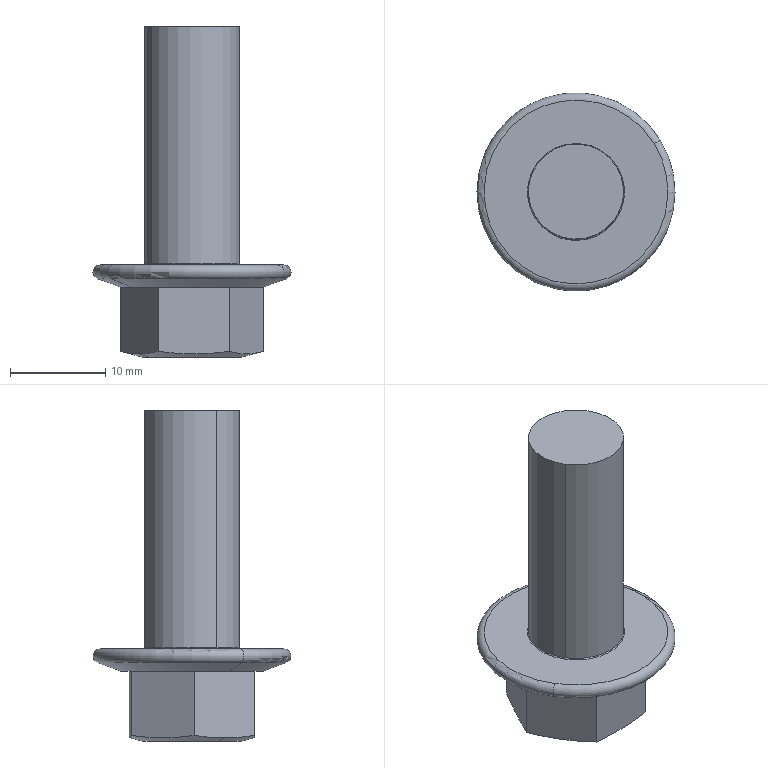Component | SolidWorks | HexFlangeBoltM10x25-10 | 1 solid | 25 faces | box 20.8 x 20.8 x 34.7 mm | volume 3718 mm3 | plane 15 | torus 4 | cone 4 | cylinder 2 | commonest cylinder face diameters 10 x2
STEP:
#1=COLOUR_RGB('',0.7922,0.8196,0.9333);
#2=FILL_AREA_STYLE_COLOUR('',#1);
#3=FILL_AREA_STYLE('',(#2));
#4=SURFACE_STYLE_FILL_AREA(#3);
#5=SURFACE_SIDE_STYLE('',(#4));
#6=SURFACE_STYLE_USAGE(.BOTH.,#5);
#7=PRESENTATION_STYLE_ASSIGNMENT((#6));
#8=CARTESIAN_POINT('',(-51.055,281.47,4.315));
#9=VERTEX_POINT('',#8);
#10=CARTESIAN_POINT('',(-51.396,281.259,4.315));
#11=VERTEX_POINT('',#10);
#12=CARTESIAN_POINT('',(-51.225,281.365,4.315));
#13=DIRECTION('',(-0.,0.,-1.));
#14=DIRECTION('',(-0.8513,-0.5247,0.));
#15=AXIS2_PLACEMENT_3D('',#12,#13,#14);
#16=CIRCLE('',#15,0.2008);
#17=EDGE_CURVE('',#9,#11,#16,.T.);
#18=ORIENTED_EDGE('',*,*,#17,.F.);
#19=CARTESIAN_POINT('',(-51.058,281.468,4.319));
#20=VERTEX_POINT('',#19);
#21=CARTESIAN_POINT('',(-51.055,281.47,4.319));
#22=DIRECTION('',(-0.5247,0.8513,0.));
#23=DIRECTION('',(-0.8513,-0.5247,0.));
#24=AXIS2_PLACEMENT_3D('',#21,#22,#23);
#25=CIRCLE('',#24,0.003937);
#26=EDGE_CURVE('',#9,#20,#25,.T.);
#27=ORIENTED_EDGE('',*,*,#26,.T.);
#28=CARTESIAN_POINT('',(-51.393,281.261,4.319));
#29=VERTEX_POINT('',#28);
#30=CARTESIAN_POINT('',(-51.225,281.365,4.319));
#31=DIRECTION('',(0.,-0.,1.));
#32=DIRECTION('',(-0.8513,-0.5247,0.));
#33=AXIS2_PLACEMENT_3D('',#30,#31,#32);
#34=CIRCLE('',#33,0.1969);
#35=EDGE_CURVE('',#29,#20,#34,.T.);
#36=ORIENTED_EDGE('',*,*,#35,.F.);
#37=CARTESIAN_POINT('',(-51.396,281.259,4.319));
#38=DIRECTION('',(0.5247,-0.8513,-0.));
#39=DIRECTION('',(0.8513,0.5247,0.));
#40=AXIS2_PLACEMENT_3D('',#37,#38,#39);
#41=CIRCLE('',#40,0.003937);
#42=EDGE_CURVE('',#11,#29,#41,.T.);
#43=ORIENTED_EDGE('',*,*,#42,.F.);
#44=EDGE_LOOP('',(#18,#27,#36,#43));
#45=FACE_OUTER_BOUND('',#44,.T.);
#46=CARTESIAN_POINT('',(-51.225,281.365,4.319));
#47=DIRECTION('',(-0.,0.,-1.));
#48=DIRECTION('',(-0.8513,-0.5247,0.));
#49=AXIS2_PLACEMENT_3D('',#46,#47,#48);
#50=TOROIDAL_SURFACE('',#49,0.2008,0.003937);
#51=ADVANCED_FACE('',(#45),#50,.F.);
#52=CARTESIAN_POINT('',(-51.051,281.472,3.933));
#53=VERTEX_POINT('',#52);
#54=CARTESIAN_POINT('',(-51.4,281.257,3.933));
#55=VERTEX_POINT('',#54);
#56=CARTESIAN_POINT('',(-51.225,281.365,3.933));
#57=DIRECTION('',(0.,-0.,1.));
#58=DIRECTION('',(0.8513,0.5247,0.));
#59=AXIS2_PLACEMENT_3D('',#56,#57,#58);
#60=CIRCLE('',#59,0.2047);
#61=EDGE_CURVE('',#53,#55,#60,.T.);
#62=ORIENTED_EDGE('',*,*,#61,.T.);
#63=CARTESIAN_POINT('',(-51.443,281.23,3.946));
#64=VERTEX_POINT('',#63);
#65=CARTESIAN_POINT('',(-51.4,281.257,3.933));
#66=DIRECTION('',(-0.8223,-0.5068,0.2588));
#67=VECTOR('',#66,39.37);
#68=LINE('',#65,#67);
#69=EDGE_CURVE('',#55,#64,#68,.T.);
#70=ORIENTED_EDGE('',*,*,#69,.T.);
#71=CARTESIAN_POINT('',(-51.521,281.356,3.957));
#72=VERTEX_POINT('',#71);
#73=CARTESIAN_POINT('',(-51.521,281.356,3.957));
#74=CARTESIAN_POINT('',(-51.495,281.314,3.951));
#75=CARTESIAN_POINT('',(-51.469,281.272,3.946));
#76=CARTESIAN_POINT('',(-51.443,281.23,3.946));
#77=B_SPLINE_CURVE_WITH_KNOTS('',3,(#73,#74,#75,#76),.UNSPECIFIED.,.F.,.F.,(4,4),(0.0185,0.02227),.UNSPECIFIED.);
#78=EDGE_CURVE('',#72,#64,#77,.T.);
#79=ORIENTED_EDGE('',*,*,#78,.F.);
#80=CARTESIAN_POINT('',(-51.38,281.616,3.957));
#81=VERTEX_POINT('',#80);
#82=CARTESIAN_POINT('',(-51.38,281.616,3.957));
#83=CARTESIAN_POINT('',(-51.404,281.573,3.95));
#84=CARTESIAN_POINT('',(-51.451,281.486,3.942));
#85=CARTESIAN_POINT('',(-51.497,281.4,3.95));
#86=CARTESIAN_POINT('',(-51.521,281.356,3.957));
#87=B_SPLINE_CURVE_WITH_KNOTS('',3,(#82,#83,#84,#85,#86),.UNSPECIFIED.,.F.,.F.,(4,1,4),(0.00000023,0.003753,0.007506),.UNSPECIFIED.);
#88=EDGE_CURVE('',#81,#72,#87,.T.);
#89=ORIENTED_EDGE('',*,*,#88,.F.);
#90=CARTESIAN_POINT('',(-51.085,281.625,3.957));
#91=VERTEX_POINT('',#90);
#92=CARTESIAN_POINT('',(-51.085,281.625,3.957));
#93=CARTESIAN_POINT('',(-51.134,281.623,3.95));
#94=CARTESIAN_POINT('',(-51.233,281.621,3.942));
#95=CARTESIAN_POINT('',(-51.331,281.618,3.95));
#96=CARTESIAN_POINT('',(-51.38,281.616,3.957));
#97=B_SPLINE_CURVE_WITH_KNOTS('',3,(#92,#93,#94,#95,#96),.UNSPECIFIED.,.F.,.F.,(4,1,4),(0.00000023,0.003753,0.007506),.UNSPECIFIED.);
#98=EDGE_CURVE('',#91,#81,#97,.T.);
#99=ORIENTED_EDGE('',*,*,#98,.F.);
#100=CARTESIAN_POINT('',(-51.008,281.499,3.946));
#101=VERTEX_POINT('',#100);
#102=CARTESIAN_POINT('',(-51.008,281.499,3.946));
#103=CARTESIAN_POINT('',(-51.033,281.541,3.946));
#104=CARTESIAN_POINT('',(-51.059,281.583,3.951));
#105=CARTESIAN_POINT('',(-51.085,281.625,3.957));
#106=B_SPLINE_CURVE_WITH_KNOTS('',3,(#102,#103,#104,#105),.UNSPECIFIED.,.F.,.F.,(4,4),(0.01018,0.01397),.UNSPECIFIED.);
#107=EDGE_CURVE('',#101,#91,#106,.T.);
#108=ORIENTED_EDGE('',*,*,#107,.F.);
#109=CARTESIAN_POINT('',(-51.051,281.472,3.933));
#110=DIRECTION('',(0.8223,0.5068,0.2588));
#111=VECTOR('',#110,39.37);
#112=LINE('',#109,#111);
#113=EDGE_CURVE('',#53,#101,#112,.T.);
#114=ORIENTED_EDGE('',*,*,#113,.F.);
#115=EDGE_LOOP('',(#62,#70,#79,#89,#99,#108,#114));
#116=FACE_OUTER_BOUND('',#115,.T.);
#117=CARTESIAN_POINT('',(-51.225,281.365,3.933));
#118=DIRECTION('',(0.,-0.,1.));
#119=DIRECTION('',(0.8513,0.5247,0.));
#120=AXIS2_PLACEMENT_3D('',#117,#118,#119);
#121=CONICAL_SURFACE('',#120,0.2047,1.309);
#122=ADVANCED_FACE('',(#116),#121,.T.);
#123=CARTESIAN_POINT('',(-51.477,281.21,4.223));
#124=VERTEX_POINT('',#123);
#125=CARTESIAN_POINT('',(-51.521,281.356,4.223));
#126=VERTEX_POINT('',#125);
#127=CARTESIAN_POINT('',(-51.225,281.365,4.223));
#128=DIRECTION('',(-0.,0.,-1.));
#129=DIRECTION('',(-0.8513,-0.5247,0.));
#130=AXIS2_PLACEMENT_3D('',#127,#128,#129);
#131=CIRCLE('',#130,0.2955);
#132=EDGE_CURVE('',#124,#126,#131,.T.);
#133=ORIENTED_EDGE('',*,*,#132,.F.);
#134=CARTESIAN_POINT('',(-51.557,281.16,4.257));
#135=VERTEX_POINT('',#134);
#136=CARTESIAN_POINT('',(-51.557,281.16,4.257));
#137=DIRECTION('',(-0.8,-0.493,0.342));
#138=VECTOR('',#137,39.37);
#139=LINE('',#136,#138);
#140=EDGE_CURVE('',#124,#135,#139,.T.);
#141=ORIENTED_EDGE('',*,*,#140,.T.);
#142=CARTESIAN_POINT('',(-50.893,281.569,4.257));
#143=VERTEX_POINT('',#142);
#144=CARTESIAN_POINT('',(-51.225,281.365,4.257));
#145=DIRECTION('',(-0.,0.,-1.));
#146=DIRECTION('',(-0.8513,-0.5247,0.));
#147=AXIS2_PLACEMENT_3D('',#144,#145,#146);
#148=CIRCLE('',#147,0.39);
#149=EDGE_CURVE('',#135,#143,#148,.T.);
#150=ORIENTED_EDGE('',*,*,#149,.T.);
#151=CARTESIAN_POINT('',(-50.974,281.52,4.223));
#152=VERTEX_POINT('',#151);
#153=CARTESIAN_POINT('',(-50.893,281.569,4.257));
#154=DIRECTION('',(0.8,0.493,0.342));
#155=VECTOR('',#154,39.37);
#156=LINE('',#153,#155);
#157=EDGE_CURVE('',#152,#143,#156,.T.);
#158=ORIENTED_EDGE('',*,*,#157,.F.);
#159=CARTESIAN_POINT('',(-51.085,281.625,4.223));
#160=VERTEX_POINT('',#159);
#161=CARTESIAN_POINT('',(-51.225,281.365,4.223));
#162=DIRECTION('',(-0.,0.,-1.));
#163=DIRECTION('',(-0.8513,-0.5247,0.));
#164=AXIS2_PLACEMENT_3D('',#161,#162,#163);
#165=CIRCLE('',#164,0.2955);
#166=EDGE_CURVE('',#160,#152,#165,.T.);
#167=ORIENTED_EDGE('',*,*,#166,.F.);
#168=CARTESIAN_POINT('',(-51.38,281.616,4.223));
#169=VERTEX_POINT('',#168);
#170=CARTESIAN_POINT('',(-51.225,281.365,4.223));
#171=DIRECTION('',(-0.,0.,-1.));
#172=DIRECTION('',(-0.8513,-0.5247,0.));
#173=AXIS2_PLACEMENT_3D('',#170,#171,#172);
#174=CIRCLE('',#173,0.2955);
#175=EDGE_CURVE('',#169,#160,#174,.T.);
#176=ORIENTED_EDGE('',*,*,#175,.F.);
#177=CARTESIAN_POINT('',(-51.225,281.365,4.223));
#178=DIRECTION('',(-0.,0.,-1.));
#179=DIRECTION('',(-0.8513,-0.5247,0.));
#180=AXIS2_PLACEMENT_3D('',#177,#178,#179);
#181=CIRCLE('',#180,0.2955);
#182=EDGE_CURVE('',#126,#169,#181,.T.);
#183=ORIENTED_EDGE('',*,*,#182,.F.);
#184=EDGE_LOOP('',(#133,#141,#150,#158,#167,#176,#183));
#185=FACE_OUTER_BOUND('',#184,.T.);
#186=CARTESIAN_POINT('',(-51.225,281.365,4.257));
#187=DIRECTION('',(0.,-0.,1.));
#188=DIRECTION('',(0.8513,0.5247,0.));
#189=AXIS2_PLACEMENT_3D('',#186,#187,#188);
#190=CONICAL_SURFACE('',#189,0.39,1.222);
#191=ADVANCED_FACE('',(#185),#190,.T.);
#192=CARTESIAN_POINT('',(-51.549,281.165,4.315));
#193=VERTEX_POINT('',#192);
#194=CARTESIAN_POINT('',(-50.902,281.564,4.315));
#195=VERTEX_POINT('',#194);
#196=CARTESIAN_POINT('',(-51.225,281.365,4.315));
#197=DIRECTION('',(-0.,0.,-1.));
#198=DIRECTION('',(-0.8513,-0.5247,0.));
#199=AXIS2_PLACEMENT_3D('',#196,#197,#198);
#200=CIRCLE('',#199,0.3799);
#201=EDGE_CURVE('',#193,#195,#200,.T.);
#202=ORIENTED_EDGE('',*,*,#201,.T.);
#203=CARTESIAN_POINT('',(-50.902,281.564,4.285));
#204=DIRECTION('',(-0.5247,0.8513,0.));
#205=DIRECTION('',(-0.8513,-0.5247,0.));
#206=AXIS2_PLACEMENT_3D('',#203,#204,#205);
#207=CIRCLE('',#206,0.02953);
#208=EDGE_CURVE('',#195,#143,#207,.T.);
#209=ORIENTED_EDGE('',*,*,#208,.T.);
#210=ORIENTED_EDGE('',*,*,#149,.F.);
#211=CARTESIAN_POINT('',(-51.549,281.165,4.285));
#212=DIRECTION('',(0.5247,-0.8513,-0.));
#213=DIRECTION('',(0.8513,0.5247,0.));
#214=AXIS2_PLACEMENT_3D('',#211,#212,#213);
#215=CIRCLE('',#214,0.02953);
#216=EDGE_CURVE('',#193,#135,#215,.T.);
#217=ORIENTED_EDGE('',*,*,#216,.F.);
#218=EDGE_LOOP('',(#202,#209,#210,#217));
#219=FACE_OUTER_BOUND('',#218,.T.);
#220=CARTESIAN_POINT('',(-51.225,281.365,4.285));
#221=DIRECTION('',(-0.,0.,-1.));
#222=DIRECTION('',(-0.8513,-0.5247,0.));
#223=AXIS2_PLACEMENT_3D('',#220,#221,#222);
#224=TOROIDAL_SURFACE('',#223,0.3799,0.02953);
#225=ADVANCED_FACE('',(#219),#224,.T.);
#226=CARTESIAN_POINT('',(-51.393,281.261,5.299));
#227=VERTEX_POINT('',#226);
#228=CARTESIAN_POINT('',(-51.058,281.468,5.299));
#229=VERTEX_POINT('',#228);
#230=CARTESIAN_POINT('',(-51.225,281.365,5.299));
#231=DIRECTION('',(-0.,0.,-1.));
#232=DIRECTION('',(-0.8513,-0.5247,0.));
#233=AXIS2_PLACEMENT_3D('',#230,#231,#232);
#234=CIRCLE('',#233,0.1969);
#235=EDGE_CURVE('',#227,#229,#234,.T.);
#236=ORIENTED_EDGE('',*,*,#235,.T.);
#237=CARTESIAN_POINT('',(-51.058,281.468,5.299));
#238=DIRECTION('',(-0.,0.,-1.));
#239=VECTOR('',#238,39.37);
#240=LINE('',#237,#239);
#241=EDGE_CURVE('',#229,#20,#240,.T.);
#242=ORIENTED_EDGE('',*,*,#241,.T.);
#243=CARTESIAN_POINT('',(-51.225,281.365,4.319));
#244=DIRECTION('',(0.,-0.,1.));
#245=DIRECTION('',(-0.8513,-0.5247,0.));
#246=AXIS2_PLACEMENT_3D('',#243,#244,#245);
#247=CIRCLE('',#246,0.1969);
#248=EDGE_CURVE('',#20,#29,#247,.T.);
#249=ORIENTED_EDGE('',*,*,#248,.T.);
#250=CARTESIAN_POINT('',(-51.393,281.261,5.299));
#251=DIRECTION('',(-0.,0.,-1.));
#252=VECTOR('',#251,39.37);
#253=LINE('',#250,#252);
#254=EDGE_CURVE('',#227,#29,#253,.T.);
#255=ORIENTED_EDGE('',*,*,#254,.F.);
#256=EDGE_LOOP('',(#236,#242,#249,#255));
#257=FACE_OUTER_BOUND('',#256,.T.);
#258=CARTESIAN_POINT('',(-51.225,281.365,5.299));
#259=DIRECTION('',(-0.,0.,-1.));
#260=DIRECTION('',(-0.8513,-0.5247,0.));
#261=AXIS2_PLACEMENT_3D('',#258,#259,#260);
#262=CYLINDRICAL_SURFACE('',#261,0.1969);
#263=ADVANCED_FACE('',(#257),#262,.T.);
#264=CARTESIAN_POINT('',(-51.225,281.365,4.315));
#265=DIRECTION('',(-0.,0.,-1.));
#266=DIRECTION('',(-0.8513,-0.5247,0.));
#267=AXIS2_PLACEMENT_3D('',#264,#265,#266);
#268=CIRCLE('',#267,0.2008);
#269=EDGE_CURVE('',#11,#9,#268,.T.);
#270=ORIENTED_EDGE('',*,*,#269,.T.);
#271=ORIENTED_EDGE('',*,*,#17,.T.);
#272=EDGE_LOOP('',(#270,#271));
#273=FACE_BOUND('',#272,.T.);
#274=ORIENTED_EDGE('',*,*,#201,.F.);
#275=CARTESIAN_POINT('',(-51.225,281.365,4.315));
#276=DIRECTION('',(-0.,0.,-1.));
#277=DIRECTION('',(-0.8513,-0.5247,0.));
#278=AXIS2_PLACEMENT_3D('',#275,#276,#277);
#279=CIRCLE('',#278,0.3799);
#280=EDGE_CURVE('',#195,#193,#279,.T.);
#281=ORIENTED_EDGE('',*,*,#280,.F.);
#282=EDGE_LOOP('',(#274,#281));
#283=FACE_OUTER_BOUND('',#282,.T.);
#284=CARTESIAN_POINT('',(-51.225,281.365,4.315));
#285=DIRECTION('',(-0.,0.,-1.));
#286=DIRECTION('',(-0.8513,-0.5247,0.));
#287=AXIS2_PLACEMENT_3D('',#284,#285,#286);
#288=PLANE('',#287);
#289=ADVANCED_FACE('',(#273,#283),#288,.F.);
#290=ORIENTED_EDGE('',*,*,#241,.F.);
#291=CARTESIAN_POINT('',(-51.225,281.365,5.299));
#292=DIRECTION('',(-0.,0.,-1.));
#293=DIRECTION('',(-0.8513,-0.5247,0.));
#294=AXIS2_PLACEMENT_3D('',#291,#292,#293);
#295=CIRCLE('',#294,0.1969);
#296=EDGE_CURVE('',#229,#227,#295,.T.);
#297=ORIENTED_EDGE('',*,*,#296,.T.);
#298=ORIENTED_EDGE('',*,*,#254,.T.);
#299=ORIENTED_EDGE('',*,*,#35,.T.);
#300=EDGE_LOOP('',(#290,#297,#298,#299));
#301=FACE_OUTER_BOUND('',#300,.T.);
#302=CARTESIAN_POINT('',(-51.225,281.365,5.299));
#303=DIRECTION('',(-0.,0.,-1.));
#304=DIRECTION('',(-0.8513,-0.5247,0.));
#305=AXIS2_PLACEMENT_3D('',#302,#303,#304);
#306=CYLINDRICAL_SURFACE('',#305,0.1969);
#307=ADVANCED_FACE('',(#301),#306,.T.);
#308=ORIENTED_EDGE('',*,*,#235,.F.);
#309=ORIENTED_EDGE('',*,*,#296,.F.);
#310=EDGE_LOOP('',(#308,#309));
#311=FACE_OUTER_BOUND('',#310,.T.);
#312=CARTESIAN_POINT('',(-51.225,281.365,5.299));
#313=DIRECTION('',(-0.,0.,-1.));
#314=DIRECTION('',(-0.8513,-0.5247,0.));
#315=AXIS2_PLACEMENT_3D('',#312,#313,#314);
#316=PLANE('',#315);
#317=ADVANCED_FACE('',(#311),#316,.F.);
#318=ORIENTED_EDGE('',*,*,#182,.T.);
#319=CARTESIAN_POINT('',(-51.521,281.356,4.223));
#320=DIRECTION('',(-0.4749,-0.88,0.));
#321=VECTOR('',#320,39.37);
#322=LINE('',#319,#321);
#323=EDGE_CURVE('',#169,#126,#322,.T.);
#324=ORIENTED_EDGE('',*,*,#323,.T.);
#325=EDGE_LOOP('',(#318,#324));
#326=FACE_OUTER_BOUND('',#325,.T.);
#327=CARTESIAN_POINT('',(-51.38,281.616,4.223));
#328=DIRECTION('',(0.,-0.,1.));
#329=DIRECTION('',(0.8513,0.5247,-0.));
#330=AXIS2_PLACEMENT_3D('',#327,#328,#329);
#331=PLANE('',#330);
#332=ADVANCED_FACE('',(#326),#331,.F.);
#333=ORIENTED_EDGE('',*,*,#175,.T.);
#334=CARTESIAN_POINT('',(-51.38,281.616,4.223));
#335=DIRECTION('',(-0.9996,-0.02872,0.));
#336=VECTOR('',#335,39.37);
#337=LINE('',#334,#336);
#338=EDGE_CURVE('',#160,#169,#337,.T.);
#339=ORIENTED_EDGE('',*,*,#338,.T.);
#340=EDGE_LOOP('',(#333,#339));
#341=FACE_OUTER_BOUND('',#340,.T.);
#342=CARTESIAN_POINT('',(-51.38,281.616,4.223));
#343=DIRECTION('',(0.,-0.,1.));
#344=DIRECTION('',(0.8513,0.5247,-0.));
#345=AXIS2_PLACEMENT_3D('',#342,#343,#344);
#346=PLANE('',#345);
#347=ADVANCED_FACE('',(#341),#346,.F.);
#348=ORIENTED_EDGE('',*,*,#166,.T.);
#349=CARTESIAN_POINT('',(-50.93,281.373,4.223));
#350=VERTEX_POINT('',#349);
#351=CARTESIAN_POINT('',(-51.225,281.365,4.223));
#352=DIRECTION('',(-0.,0.,-1.));
#353=DIRECTION('',(-0.8513,-0.5247,0.));
#354=AXIS2_PLACEMENT_3D('',#351,#352,#353);
#355=CIRCLE('',#354,0.2955);
#356=EDGE_CURVE('',#152,#350,#355,.T.);
#357=ORIENTED_EDGE('',*,*,#356,.T.);
#358=CARTESIAN_POINT('',(-51.085,281.625,4.223));
#359=DIRECTION('',(-0.5247,0.8513,0.));
#360=VECTOR('',#359,39.37);
#361=LINE('',#358,#360);
#362=EDGE_CURVE('',#350,#160,#361,.T.);
#363=ORIENTED_EDGE('',*,*,#362,.T.);
#364=EDGE_LOOP('',(#348,#357,#363));
#365=FACE_OUTER_BOUND('',#364,.T.);
#366=CARTESIAN_POINT('',(-51.38,281.616,4.223));
#367=DIRECTION('',(0.,-0.,1.));
#368=DIRECTION('',(0.8513,0.5247,-0.));
#369=AXIS2_PLACEMENT_3D('',#366,#367,#368);
#370=PLANE('',#369);
#371=ADVANCED_FACE('',(#365),#370,.F.);
#372=CARTESIAN_POINT('',(-51.07,281.113,4.223));
#373=VERTEX_POINT('',#372);
#374=CARTESIAN_POINT('',(-51.225,281.365,4.223));
#375=DIRECTION('',(-0.,0.,-1.));
#376=DIRECTION('',(-0.8513,-0.5247,0.));
#377=AXIS2_PLACEMENT_3D('',#374,#375,#376);
#378=CIRCLE('',#377,0.2955);
#379=EDGE_CURVE('',#350,#373,#378,.T.);
#380=ORIENTED_EDGE('',*,*,#379,.T.);
#381=CARTESIAN_POINT('',(-50.93,281.373,4.223));
#382=DIRECTION('',(0.4749,0.88,-0.));
#383=VECTOR('',#382,39.37);
#384=LINE('',#381,#383);
#385=EDGE_CURVE('',#373,#350,#384,.T.);
#386=ORIENTED_EDGE('',*,*,#385,.T.);
#387=EDGE_LOOP('',(#380,#386));
#388=FACE_OUTER_BOUND('',#387,.T.);
#389=CARTESIAN_POINT('',(-51.38,281.616,4.223));
#390=DIRECTION('',(0.,-0.,1.));
#391=DIRECTION('',(0.8513,0.5247,-0.));
#392=AXIS2_PLACEMENT_3D('',#389,#390,#391);
#393=PLANE('',#392);
#394=ADVANCED_FACE('',(#388),#393,.F.);
#395=CARTESIAN_POINT('',(-51.366,281.105,4.223));
#396=VERTEX_POINT('',#395);
#397=CARTESIAN_POINT('',(-51.225,281.365,4.223));
#398=DIRECTION('',(-0.,0.,-1.));
#399=DIRECTION('',(-0.8513,-0.5247,0.));
#400=AXIS2_PLACEMENT_3D('',#397,#398,#399);
#401=CIRCLE('',#400,0.2955);
#402=EDGE_CURVE('',#373,#396,#401,.T.);
#403=ORIENTED_EDGE('',*,*,#402,.T.);
#404=CARTESIAN_POINT('',(-51.07,281.113,4.223));
#405=DIRECTION('',(0.9996,0.02872,-0.));
#406=VECTOR('',#405,39.37);
#407=LINE('',#404,#406);
#408=EDGE_CURVE('',#396,#373,#407,.T.);
#409=ORIENTED_EDGE('',*,*,#408,.T.);
#410=EDGE_LOOP('',(#403,#409));
#411=FACE_OUTER_BOUND('',#410,.T.);
#412=CARTESIAN_POINT('',(-51.38,281.616,4.223));
#413=DIRECTION('',(0.,-0.,1.));
#414=DIRECTION('',(0.8513,0.5247,-0.));
#415=AXIS2_PLACEMENT_3D('',#412,#413,#414);
#416=PLANE('',#415);
#417=ADVANCED_FACE('',(#411),#416,.F.);
#418=CARTESIAN_POINT('',(-51.225,281.365,4.223));
#419=DIRECTION('',(-0.,0.,-1.));
#420=DIRECTION('',(-0.8513,-0.5247,0.));
#421=AXIS2_PLACEMENT_3D('',#418,#419,#420);
#422=CIRCLE('',#421,0.2955);
#423=EDGE_CURVE('',#396,#124,#422,.T.);
#424=ORIENTED_EDGE('',*,*,#423,.T.);
#425=ORIENTED_EDGE('',*,*,#132,.T.);
#426=CARTESIAN_POINT('',(-51.366,281.105,4.223));
#427=DIRECTION('',(0.5247,-0.8513,-0.));
#428=VECTOR('',#427,39.37);
#429=LINE('',#426,#428);
#430=EDGE_CURVE('',#126,#396,#429,.T.);
#431=ORIENTED_EDGE('',*,*,#430,.T.);
#432=EDGE_LOOP('',(#424,#425,#431));
#433=FACE_OUTER_BOUND('',#432,.T.);
#434=CARTESIAN_POINT('',(-51.38,281.616,4.223));
#435=DIRECTION('',(0.,-0.,1.));
#436=DIRECTION('',(0.8513,0.5247,-0.));
#437=AXIS2_PLACEMENT_3D('',#434,#435,#436);
#438=PLANE('',#437);
#439=ADVANCED_FACE('',(#433),#438,.F.);
#440=ORIENTED_EDGE('',*,*,#208,.F.);
#441=ORIENTED_EDGE('',*,*,#280,.T.);
#442=ORIENTED_EDGE('',*,*,#216,.T.);
#443=CARTESIAN_POINT('',(-51.225,281.365,4.257));
#444=DIRECTION('',(-0.,0.,-1.));
#445=DIRECTION('',(-0.8513,-0.5247,0.));
#446=AXIS2_PLACEMENT_3D('',#443,#444,#445);
#447=CIRCLE('',#446,0.39);
#448=EDGE_CURVE('',#143,#135,#447,.T.);
#449=ORIENTED_EDGE('',*,*,#448,.F.);
#450=EDGE_LOOP('',(#440,#441,#442,#449));
#451=FACE_OUTER_BOUND('',#450,.T.);
#452=CARTESIAN_POINT('',(-51.225,281.365,4.285));
#453=DIRECTION('',(-0.,0.,-1.));
#454=DIRECTION('',(-0.8513,-0.5247,0.));
#455=AXIS2_PLACEMENT_3D('',#452,#453,#454);
#456=TOROIDAL_SURFACE('',#455,0.3799,0.02953);
#457=ADVANCED_FACE('',(#451),#456,.T.);
#458=ORIENTED_EDGE('',*,*,#140,.F.);
#459=ORIENTED_EDGE('',*,*,#423,.F.);
#460=ORIENTED_EDGE('',*,*,#402,.F.);
#461=ORIENTED_EDGE('',*,*,#379,.F.);
#462=ORIENTED_EDGE('',*,*,#356,.F.);
#463=ORIENTED_EDGE('',*,*,#157,.T.);
#464=ORIENTED_EDGE('',*,*,#448,.T.);
#465=EDGE_LOOP('',(#458,#459,#460,#461,#462,#463,#464));
#466=FACE_OUTER_BOUND('',#465,.T.);
#467=CARTESIAN_POINT('',(-51.225,281.365,4.257));
#468=DIRECTION('',(0.,-0.,1.));
#469=DIRECTION('',(0.8513,0.5247,0.));
#470=AXIS2_PLACEMENT_3D('',#467,#468,#469);
#471=CONICAL_SURFACE('',#470,0.39,1.222);
#472=ADVANCED_FACE('',(#466),#471,.T.);
#473=CARTESIAN_POINT('',(-51.521,281.356,3.933));
#474=DIRECTION('',(0.,-0.,1.));
#475=VECTOR('',#474,39.37);
#476=LINE('',#473,#475);
#477=EDGE_CURVE('',#72,#126,#476,.T.);
#478=ORIENTED_EDGE('',*,*,#477,.F.);
#479=ORIENTED_EDGE('',*,*,#78,.T.);
#480=CARTESIAN_POINT('',(-51.366,281.105,3.957));
#481=VERTEX_POINT('',#480);
#482=CARTESIAN_POINT('',(-51.443,281.23,3.946));
#483=CARTESIAN_POINT('',(-51.43,281.21,3.946));
#484=CARTESIAN_POINT('',(-51.418,281.189,3.947));
#485=CARTESIAN_POINT('',(-51.392,281.147,3.951));
#486=CARTESIAN_POINT('',(-51.379,281.126,3.954));
#487=CARTESIAN_POINT('',(-51.366,281.105,3.957));
#488=B_SPLINE_CURVE_WITH_KNOTS('',3,(#482,#483,#484,#485,#486,#487),.UNSPECIFIED.,.F.,.F.,(4,2,4),(0.02227,0.02416,0.02604),.UNSPECIFIED.);
#489=EDGE_CURVE('',#64,#481,#488,.T.);
#490=ORIENTED_EDGE('',*,*,#489,.T.);
#491=CARTESIAN_POINT('',(-51.366,281.105,3.933));
#492=DIRECTION('',(0.,-0.,1.));
#493=VECTOR('',#492,39.37);
#494=LINE('',#491,#493);
#495=EDGE_CURVE('',#481,#396,#494,.T.);
#496=ORIENTED_EDGE('',*,*,#495,.T.);
#497=ORIENTED_EDGE('',*,*,#430,.F.);
#498=EDGE_LOOP('',(#478,#479,#490,#496,#497));
#499=FACE_OUTER_BOUND('',#498,.T.);
#500=CARTESIAN_POINT('',(-51.366,281.105,3.933));
#501=DIRECTION('',(0.8513,0.5247,-0.));
#502=DIRECTION('',(0.5247,-0.8513,-0.));
#503=AXIS2_PLACEMENT_3D('',#500,#501,#502);
#504=PLANE('',#503);
#505=ADVANCED_FACE('',(#499),#504,.F.);
#506=ORIENTED_EDGE('',*,*,#495,.F.);
#507=CARTESIAN_POINT('',(-51.07,281.113,3.957));
#508=VERTEX_POINT('',#507);
#509=CARTESIAN_POINT('',(-51.366,281.105,3.957));
#510=CARTESIAN_POINT('',(-51.317,281.106,3.95));
#511=CARTESIAN_POINT('',(-51.218,281.109,3.942));
#512=CARTESIAN_POINT('',(-51.12,281.112,3.95));
#513=CARTESIAN_POINT('',(-51.07,281.113,3.957));
#514=B_SPLINE_CURVE_WITH_KNOTS('',3,(#509,#510,#511,#512,#513),.UNSPECIFIED.,.F.,.F.,(4,1,4),(0.00000023,0.003753,0.007506),.UNSPECIFIED.);
#515=EDGE_CURVE('',#481,#508,#514,.T.);
#516=ORIENTED_EDGE('',*,*,#515,.T.);
#517=CARTESIAN_POINT('',(-51.07,281.113,3.933));
#518=DIRECTION('',(0.,-0.,1.));
#519=VECTOR('',#518,39.37);
#520=LINE('',#517,#519);
#521=EDGE_CURVE('',#508,#373,#520,.T.);
#522=ORIENTED_EDGE('',*,*,#521,.T.);
#523=ORIENTED_EDGE('',*,*,#408,.F.);
#524=EDGE_LOOP('',(#506,#516,#522,#523));
#525=FACE_OUTER_BOUND('',#524,.T.);
#526=CARTESIAN_POINT('',(-51.07,281.113,3.933));
#527=DIRECTION('',(-0.02872,0.9996,0.));
#528=DIRECTION('',(0.9996,0.02872,-0.));
#529=AXIS2_PLACEMENT_3D('',#526,#527,#528);
#530=PLANE('',#529);
#531=ADVANCED_FACE('',(#525),#530,.F.);
#532=ORIENTED_EDGE('',*,*,#521,.F.);
#533=CARTESIAN_POINT('',(-50.93,281.373,3.957));
#534=VERTEX_POINT('',#533);
#535=CARTESIAN_POINT('',(-51.07,281.113,3.957));
#536=CARTESIAN_POINT('',(-51.047,281.157,3.95));
#537=CARTESIAN_POINT('',(-51.,281.243,3.942));
#538=CARTESIAN_POINT('',(-50.953,281.33,3.95));
#539=CARTESIAN_POINT('',(-50.93,281.373,3.957));
#540=B_SPLINE_CURVE_WITH_KNOTS('',3,(#535,#536,#537,#538,#539),.UNSPECIFIED.,.F.,.F.,(4,1,4),(0.00000023,0.003753,0.007506),.UNSPECIFIED.);
#541=EDGE_CURVE('',#508,#534,#540,.T.);
#542=ORIENTED_EDGE('',*,*,#541,.T.);
#543=CARTESIAN_POINT('',(-50.93,281.373,3.933));
#544=DIRECTION('',(0.,-0.,1.));
#545=VECTOR('',#544,39.37);
#546=LINE('',#543,#545);
#547=EDGE_CURVE('',#534,#350,#546,.T.);
#548=ORIENTED_EDGE('',*,*,#547,.T.);
#549=ORIENTED_EDGE('',*,*,#385,.F.);
#550=EDGE_LOOP('',(#532,#542,#548,#549));
#551=FACE_OUTER_BOUND('',#550,.T.);
#552=CARTESIAN_POINT('',(-50.93,281.373,3.933));
#553=DIRECTION('',(-0.88,0.4749,0.));
#554=DIRECTION('',(0.4749,0.88,-0.));
#555=AXIS2_PLACEMENT_3D('',#552,#553,#554);
#556=PLANE('',#555);
#557=ADVANCED_FACE('',(#551),#556,.F.);
#558=ORIENTED_EDGE('',*,*,#547,.F.);
#559=CARTESIAN_POINT('',(-50.93,281.373,3.957));
#560=CARTESIAN_POINT('',(-50.943,281.394,3.954));
#561=CARTESIAN_POINT('',(-50.956,281.415,3.951));
#562=CARTESIAN_POINT('',(-50.982,281.457,3.947));
#563=CARTESIAN_POINT('',(-50.995,281.478,3.946));
#564=CARTESIAN_POINT('',(-51.008,281.499,3.946));
#565=B_SPLINE_CURVE_WITH_KNOTS('',3,(#559,#560,#561,#562,#563,#564),.UNSPECIFIED.,.F.,.F.,(4,2,4),(0.006413,0.008299,0.01018),.UNSPECIFIED.);
#566=EDGE_CURVE('',#534,#101,#565,.T.);
#567=ORIENTED_EDGE('',*,*,#566,.T.);
#568=ORIENTED_EDGE('',*,*,#107,.T.);
#569=CARTESIAN_POINT('',(-51.085,281.625,3.933));
#570=DIRECTION('',(0.,-0.,1.));
#571=VECTOR('',#570,39.37);
#572=LINE('',#569,#571);
#573=EDGE_CURVE('',#91,#160,#572,.T.);
#574=ORIENTED_EDGE('',*,*,#573,.T.);
#575=ORIENTED_EDGE('',*,*,#362,.F.);
#576=EDGE_LOOP('',(#558,#567,#568,#574,#575));
#577=FACE_OUTER_BOUND('',#576,.T.);
#578=CARTESIAN_POINT('',(-51.085,281.625,3.933));
#579=DIRECTION('',(-0.8513,-0.5247,0.));
#580=DIRECTION('',(0.,-0.,1.));
#581=AXIS2_PLACEMENT_3D('',#578,#579,#580);
#582=PLANE('',#581);
#583=ADVANCED_FACE('',(#577),#582,.F.);
#584=ORIENTED_EDGE('',*,*,#573,.F.);
#585=ORIENTED_EDGE('',*,*,#98,.T.);
#586=CARTESIAN_POINT('',(-51.38,281.616,3.933));
#587=DIRECTION('',(0.,-0.,1.));
#588=VECTOR('',#587,39.37);
#589=LINE('',#586,#588);
#590=EDGE_CURVE('',#81,#169,#589,.T.);
#591=ORIENTED_EDGE('',*,*,#590,.T.);
#592=ORIENTED_EDGE('',*,*,#338,.F.);
#593=EDGE_LOOP('',(#584,#585,#591,#592));
#594=FACE_OUTER_BOUND('',#593,.T.);
#595=CARTESIAN_POINT('',(-51.38,281.616,3.933));
#596=DIRECTION('',(0.02872,-0.9996,-0.));
#597=DIRECTION('',(-0.9996,-0.02872,0.));
#598=AXIS2_PLACEMENT_3D('',#595,#596,#597);
#599=PLANE('',#598);
#600=ADVANCED_FACE('',(#594),#599,.F.);
#601=ORIENTED_EDGE('',*,*,#590,.F.);
#602=ORIENTED_EDGE('',*,*,#88,.T.);
#603=ORIENTED_EDGE('',*,*,#477,.T.);
#604=ORIENTED_EDGE('',*,*,#323,.F.);
#605=EDGE_LOOP('',(#601,#602,#603,#604));
#606=FACE_OUTER_BOUND('',#605,.T.);
#607=CARTESIAN_POINT('',(-51.521,281.356,3.933));
#608=DIRECTION('',(0.88,-0.4749,-0.));
#609=DIRECTION('',(-0.4749,-0.88,0.));
#610=AXIS2_PLACEMENT_3D('',#607,#608,#609);
#611=PLANE('',#610);
#612=ADVANCED_FACE('',(#606),#611,.F.);
#613=ORIENTED_EDGE('',*,*,#69,.F.);
#614=CARTESIAN_POINT('',(-51.225,281.365,3.933));
#615=DIRECTION('',(0.,-0.,1.));
#616=DIRECTION('',(0.8513,0.5247,0.));
#617=AXIS2_PLACEMENT_3D('',#614,#615,#616);
#618=CIRCLE('',#617,0.2047);
#619=EDGE_CURVE('',#55,#53,#618,.T.);
#620=ORIENTED_EDGE('',*,*,#619,.T.);
#621=ORIENTED_EDGE('',*,*,#113,.T.);
#622=ORIENTED_EDGE('',*,*,#566,.F.);
#623=ORIENTED_EDGE('',*,*,#541,.F.);
#624=ORIENTED_EDGE('',*,*,#515,.F.);
#625=ORIENTED_EDGE('',*,*,#489,.F.);
#626=EDGE_LOOP('',(#613,#620,#621,#622,#623,#624,#625));
#627=FACE_OUTER_BOUND('',#626,.T.);
#628=CARTESIAN_POINT('',(-51.225,281.365,3.933));
#629=DIRECTION('',(0.,-0.,1.));
#630=DIRECTION('',(0.8513,0.5247,0.));
#631=AXIS2_PLACEMENT_3D('',#628,#629,#630);
#632=CONICAL_SURFACE('',#631,0.2047,1.309);
#633=ADVANCED_FACE('',(#627),#632,.T.);
#634=ORIENTED_EDGE('',*,*,#61,.F.);
#635=ORIENTED_EDGE('',*,*,#619,.F.);
#636=EDGE_LOOP('',(#634,#635));
#637=FACE_OUTER_BOUND('',#636,.T.);
#638=CARTESIAN_POINT('',(-51.225,281.365,3.933));
#639=DIRECTION('',(-0.,0.,-1.));
#640=DIRECTION('',(-0.8513,-0.5247,0.));
#641=AXIS2_PLACEMENT_3D('',#638,#639,#640);
#642=PLANE('',#641);
#643=ADVANCED_FACE('',(#637),#642,.T.);
#644=ORIENTED_EDGE('',*,*,#26,.F.);
#645=ORIENTED_EDGE('',*,*,#269,.F.);
#646=ORIENTED_EDGE('',*,*,#42,.T.);
#647=ORIENTED_EDGE('',*,*,#248,.F.);
#648=EDGE_LOOP('',(#644,#645,#646,#647));
#649=FACE_OUTER_BOUND('',#648,.T.);
#650=CARTESIAN_POINT('',(-51.225,281.365,4.319));
#651=DIRECTION('',(-0.,0.,-1.));
#652=DIRECTION('',(-0.8513,-0.5247,0.));
#653=AXIS2_PLACEMENT_3D('',#650,#651,#652);
#654=TOROIDAL_SURFACE('',#653,0.2008,0.003937);
#655=ADVANCED_FACE('',(#649),#654,.F.);
#656=CLOSED_SHELL('',(#51,#122,#191,#225,#263,#289,#307,#317,#332,#347,#371,#394,#417,#439,#457,#472,#505,#531,#557,#583,#600,#612,#633,#643,#655));
#657=MANIFOLD_SOLID_BREP('',#656);
#658=STYLED_ITEM('',(#7),#657);
#659=PRESENTATION_LAYER_ASSIGNMENT('','',(#658));
#660=CARTESIAN_POINT('',(0.,0.,0.));
#661=DIRECTION('',(0.,0.,1.));
#662=DIRECTION('',(1.,0.,0.));
#663=AXIS2_PLACEMENT_3D('',#660,#661,#662);
#664=(LENGTH_UNIT()NAMED_UNIT(*)SI_UNIT($,.METRE.));
#665=LENGTH_MEASURE_WITH_UNIT(LENGTH_MEASURE(0.0254),#664);
#666=DIMENSIONAL_EXPONENTS(1.,0.,0.,0.,0.,0.,0.);
#667=(CONVERSION_BASED_UNIT('',#665)LENGTH_UNIT()NAMED_UNIT(#666));
#668=UNCERTAINTY_MEASURE_WITH_UNIT(LENGTH_MEASURE(0.00001),#667,'','');
#669=(NAMED_UNIT(*)PLANE_ANGLE_UNIT()SI_UNIT($,.RADIAN.));
#670=(NAMED_UNIT(*)SI_UNIT($,.STERADIAN.)SOLID_ANGLE_UNIT());
#671=(GEOMETRIC_REPRESENTATION_CONTEXT(3)GLOBAL_UNCERTAINTY_ASSIGNED_CONTEXT((#668))GLOBAL_UNIT_ASSIGNED_CONTEXT((#667,#669,#670))REPRESENTATION_CONTEXT('',''));
#672=ADVANCED_BREP_SHAPE_REPRESENTATION('',(#657,#663),#671);
#673=(LENGTH_UNIT()NAMED_UNIT(*)SI_UNIT($,.METRE.));
#674=LENGTH_MEASURE_WITH_UNIT(LENGTH_MEASURE(0.0254),#673);
#675=DIMENSIONAL_EXPONENTS(1.,0.,0.,0.,0.,0.,0.);
#676=(CONVERSION_BASED_UNIT('',#674)LENGTH_UNIT()NAMED_UNIT(#675));
#677=UNCERTAINTY_MEASURE_WITH_UNIT(LENGTH_MEASURE(0.00001),#676,'','');
#678=(NAMED_UNIT(*)PLANE_ANGLE_UNIT()SI_UNIT($,.RADIAN.));
#679=(NAMED_UNIT(*)SI_UNIT($,.STERADIAN.)SOLID_ANGLE_UNIT());
#680=(GEOMETRIC_REPRESENTATION_CONTEXT(3)GLOBAL_UNCERTAINTY_ASSIGNED_CONTEXT((#677))GLOBAL_UNIT_ASSIGNED_CONTEXT((#676,#678,#679))REPRESENTATION_CONTEXT('',''));
#681=MECHANICAL_DESIGN_GEOMETRIC_PRESENTATION_REPRESENTATION('',(#658),#680);